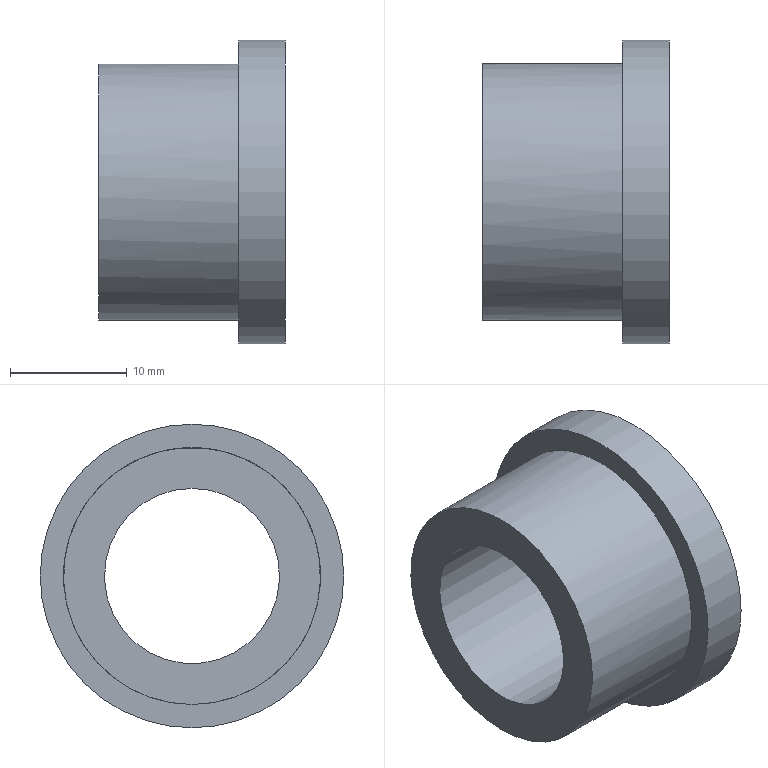Component | NX | LOCATING_BUSH | 1 solid | 6 faces | box 16 x 26 x 26 mm | volume 3858 mm3 | plane 3 | cylinder 3 | commonest cylinder face diameters 22 x1 26 x1 15 x1
STEP:
#1=CARTESIAN_POINT('',(0.,0.,0.));
#2=DIRECTION('',(0.,0.,1.));
#3=DIRECTION('',(1.,0.,0.));
#4=AXIS2_PLACEMENT_3D('',#1,#2,#3);
#5=CARTESIAN_POINT('',(-30.772,-17.527,-251.219));
#6=VERTEX_POINT('',#5);
#7=CARTESIAN_POINT('',(-30.772,-17.527,-258.719));
#8=DIRECTION('',(-1.,0.,0.));
#9=DIRECTION('',(0.,0.,1.));
#10=AXIS2_PLACEMENT_3D('',#7,#8,#9);
#11=CIRCLE('',#10,7.5);
#12=CARTESIAN_POINT('',(-30.772,-17.527,-258.719));
#13=DIRECTION('',(-1.,0.,0.));
#14=DIRECTION('',(0.,0.,1.));
#15=AXIS2_PLACEMENT_3D('',#12,#13,#14);
#16=PLANE('',#15);
#17=CARTESIAN_POINT('',(0.,0.));
#18=DIRECTION('',(1.,0.));
#19=AXIS2_PLACEMENT_2D('',#17,#18);
#20=CIRCLE('',#19,7.5);
#21=(GEOMETRIC_REPRESENTATION_CONTEXT(2)PARAMETRIC_REPRESENTATION_CONTEXT()REPRESENTATION_CONTEXT('',''));
#22=DEFINITIONAL_REPRESENTATION('',(#20),#21);
#23=PCURVE('',#16,#22);
#24=CARTESIAN_POINT('',(-14.772,-17.527,-258.719));
#25=DIRECTION('',(-1.,0.,0.));
#26=DIRECTION('',(0.,0.,1.));
#27=AXIS2_PLACEMENT_3D('',#24,#25,#26);
#28=CYLINDRICAL_SURFACE('',#27,7.5);
#29=CARTESIAN_POINT('',(0.,16.));
#30=DIRECTION('',(1.,0.));
#31=VECTOR('',#30,1.);
#32=LINE('',#29,#31);
#33=(GEOMETRIC_REPRESENTATION_CONTEXT(2)PARAMETRIC_REPRESENTATION_CONTEXT()REPRESENTATION_CONTEXT('',''));
#34=DEFINITIONAL_REPRESENTATION('',(#32),#33);
#35=PCURVE('',#28,#34);
#36=SURFACE_CURVE('',#11,(#23,#35),.PCURVE_S1.);
#37=EDGE_CURVE('',#6,#6,#36,.T.);
#38=ORIENTED_EDGE('',*,*,#37,.F.);
#39=EDGE_LOOP('',(#38));
#40=FACE_BOUND('',#39,.T.);
#41=CARTESIAN_POINT('',(-30.772,-17.527,-269.719));
#42=VERTEX_POINT('',#41);
#43=CARTESIAN_POINT('',(-30.772,-17.527,-258.719));
#44=DIRECTION('',(1.,0.,0.));
#45=DIRECTION('',(0.,0.,-1.));
#46=AXIS2_PLACEMENT_3D('',#43,#44,#45);
#47=CIRCLE('',#46,11.);
#48=CARTESIAN_POINT('',(-11.,0.));
#49=CARTESIAN_POINT('',(-11.,19.053));
#50=CARTESIAN_POINT('',(5.5,9.526));
#51=CARTESIAN_POINT('',(22.,0.));
#52=CARTESIAN_POINT('',(5.5,-9.526));
#53=CARTESIAN_POINT('',(-11.,-19.053));
#54=CARTESIAN_POINT('',(-11.,0.));
#55=(BOUNDED_CURVE()B_SPLINE_CURVE(2,(#48,#49,#50,#51,#52,#53,#54),.UNSPECIFIED.,.T.,.F.)B_SPLINE_CURVE_WITH_KNOTS((1,2,2,2,2,1),(-2.094,0.,2.094,4.189,6.283,8.378),.UNSPECIFIED.)CURVE()GEOMETRIC_REPRESENTATION_ITEM()RATIONAL_B_SPLINE_CURVE((1.,0.5,1.,0.5,1.,0.5,1.))REPRESENTATION_ITEM(''));
#56=(GEOMETRIC_REPRESENTATION_CONTEXT(2)PARAMETRIC_REPRESENTATION_CONTEXT()REPRESENTATION_CONTEXT('',''));
#57=DEFINITIONAL_REPRESENTATION('',(#55),#56);
#58=PCURVE('',#16,#57);
#59=CARTESIAN_POINT('',(-30.772,-17.527,-258.719));
#60=DIRECTION('',(1.,0.,0.));
#61=DIRECTION('',(0.,0.,-1.));
#62=AXIS2_PLACEMENT_3D('',#59,#60,#61);
#63=CYLINDRICAL_SURFACE('',#62,11.);
#64=CARTESIAN_POINT('',(0.,0.));
#65=DIRECTION('',(1.,0.));
#66=VECTOR('',#65,1.);
#67=LINE('',#64,#66);
#68=(GEOMETRIC_REPRESENTATION_CONTEXT(2)PARAMETRIC_REPRESENTATION_CONTEXT()REPRESENTATION_CONTEXT('',''));
#69=DEFINITIONAL_REPRESENTATION('',(#67),#68);
#70=PCURVE('',#63,#69);
#71=SURFACE_CURVE('',#47,(#58,#70),.PCURVE_S1.);
#72=EDGE_CURVE('',#42,#42,#71,.T.);
#73=ORIENTED_EDGE('',*,*,#72,.F.);
#74=EDGE_LOOP('',(#73));
#75=FACE_BOUND('',#74,.T.);
#76=ADVANCED_FACE('',(#40,#75),#16,.T.);
#77=CARTESIAN_POINT('',(-18.772,-17.527,-269.719));
#78=VERTEX_POINT('',#77);
#79=CARTESIAN_POINT('',(-18.772,-17.527,-247.719));
#80=VERTEX_POINT('',#79);
#81=CARTESIAN_POINT('',(-18.772,-17.527,-258.719));
#82=DIRECTION('',(1.,0.,0.));
#83=DIRECTION('',(0.,0.,1.));
#84=AXIS2_PLACEMENT_3D('',#81,#82,#83);
#85=CIRCLE('',#84,11.);
#86=CARTESIAN_POINT('',(-3.142,12.));
#87=DIRECTION('',(1.,0.));
#88=VECTOR('',#87,1.);
#89=LINE('',#86,#88);
#90=(GEOMETRIC_REPRESENTATION_CONTEXT(2)PARAMETRIC_REPRESENTATION_CONTEXT()REPRESENTATION_CONTEXT('',''));
#91=DEFINITIONAL_REPRESENTATION('',(#89),#90);
#92=PCURVE('',#63,#91);
#93=CARTESIAN_POINT('',(-18.772,-17.527,-258.719));
#94=DIRECTION('',(-1.,0.,0.));
#95=DIRECTION('',(0.,0.,1.));
#96=AXIS2_PLACEMENT_3D('',#93,#94,#95);
#97=PLANE('',#96);
#98=CARTESIAN_POINT('',(11.,0.));
#99=CARTESIAN_POINT('',(11.,-19.053));
#100=CARTESIAN_POINT('',(-5.5,-9.526));
#101=CARTESIAN_POINT('',(-22.,-0.));
#102=CARTESIAN_POINT('',(-5.5,9.526));
#103=CARTESIAN_POINT('',(11.,19.053));
#104=CARTESIAN_POINT('',(11.,0.));
#105=(BOUNDED_CURVE()B_SPLINE_CURVE(2,(#98,#99,#100,#101,#102,#103,#104),.UNSPECIFIED.,.T.,.F.)B_SPLINE_CURVE_WITH_KNOTS((1,2,2,2,2,1),(-2.094,0.,2.094,4.189,6.283,8.378),.UNSPECIFIED.)CURVE()GEOMETRIC_REPRESENTATION_ITEM()RATIONAL_B_SPLINE_CURVE((1.,0.5,1.,0.5,1.,0.5,1.))REPRESENTATION_ITEM(''));
#106=(GEOMETRIC_REPRESENTATION_CONTEXT(2)PARAMETRIC_REPRESENTATION_CONTEXT()REPRESENTATION_CONTEXT('',''));
#107=DEFINITIONAL_REPRESENTATION('',(#105),#106);
#108=PCURVE('',#97,#107);
#109=SURFACE_CURVE('',#85,(#92,#108),.PCURVE_S1.);
#110=EDGE_CURVE('',#78,#80,#109,.T.);
#111=ORIENTED_EDGE('',*,*,#110,.F.);
#112=CARTESIAN_POINT('',(-30.772,-17.527,-269.719));
#113=CARTESIAN_POINT('',(-18.772,-17.527,-269.719));
#114=B_SPLINE_CURVE_WITH_KNOTS('',1,(#112,#113),.UNSPECIFIED.,.F.,.F.,(2,2),(0.,12.),.PIECEWISE_BEZIER_KNOTS.);
#115=CARTESIAN_POINT('',(0.,0.));
#116=DIRECTION('',(0.,1.));
#117=VECTOR('',#116,1.);
#118=LINE('',#115,#117);
#119=(GEOMETRIC_REPRESENTATION_CONTEXT(2)PARAMETRIC_REPRESENTATION_CONTEXT()REPRESENTATION_CONTEXT('',''));
#120=DEFINITIONAL_REPRESENTATION('',(#118),#119);
#121=PCURVE('',#63,#120);
#122=CARTESIAN_POINT('',(6.283,0.));
#123=DIRECTION('',(0.,1.));
#124=VECTOR('',#123,1.);
#125=LINE('',#122,#124);
#126=(GEOMETRIC_REPRESENTATION_CONTEXT(2)PARAMETRIC_REPRESENTATION_CONTEXT()REPRESENTATION_CONTEXT('',''));
#127=DEFINITIONAL_REPRESENTATION('',(#125),#126);
#128=PCURVE('',#63,#127);
#129=SEAM_CURVE('',#114,(#121,#128),.PCURVE_S1.);
#130=EDGE_CURVE('',#42,#78,#129,.T.);
#131=ORIENTED_EDGE('',*,*,#130,.F.);
#132=ORIENTED_EDGE('',*,*,#72,.T.);
#133=ORIENTED_EDGE('',*,*,#130,.T.);
#134=CARTESIAN_POINT('',(-18.772,-17.527,-258.719));
#135=DIRECTION('',(1.,0.,0.));
#136=DIRECTION('',(0.,0.,1.));
#137=AXIS2_PLACEMENT_3D('',#134,#135,#136);
#138=CIRCLE('',#137,11.);
#139=CARTESIAN_POINT('',(3.142,12.));
#140=DIRECTION('',(1.,0.));
#141=VECTOR('',#140,1.);
#142=LINE('',#139,#141);
#143=(GEOMETRIC_REPRESENTATION_CONTEXT(2)PARAMETRIC_REPRESENTATION_CONTEXT()REPRESENTATION_CONTEXT('',''));
#144=DEFINITIONAL_REPRESENTATION('',(#142),#143);
#145=PCURVE('',#63,#144);
#146=CARTESIAN_POINT('',(11.,0.));
#147=CARTESIAN_POINT('',(11.,-19.053));
#148=CARTESIAN_POINT('',(-5.5,-9.526));
#149=CARTESIAN_POINT('',(-22.,-0.));
#150=CARTESIAN_POINT('',(-5.5,9.526));
#151=CARTESIAN_POINT('',(11.,19.053));
#152=CARTESIAN_POINT('',(11.,0.));
#153=(BOUNDED_CURVE()B_SPLINE_CURVE(2,(#146,#147,#148,#149,#150,#151,#152),.UNSPECIFIED.,.T.,.F.)B_SPLINE_CURVE_WITH_KNOTS((1,2,2,2,2,1),(-2.094,0.,2.094,4.189,6.283,8.378),.UNSPECIFIED.)CURVE()GEOMETRIC_REPRESENTATION_ITEM()RATIONAL_B_SPLINE_CURVE((1.,0.5,1.,0.5,1.,0.5,1.))REPRESENTATION_ITEM(''));
#154=(GEOMETRIC_REPRESENTATION_CONTEXT(2)PARAMETRIC_REPRESENTATION_CONTEXT()REPRESENTATION_CONTEXT('',''));
#155=DEFINITIONAL_REPRESENTATION('',(#153),#154);
#156=PCURVE('',#97,#155);
#157=SURFACE_CURVE('',#138,(#145,#156),.PCURVE_S1.);
#158=EDGE_CURVE('',#80,#78,#157,.T.);
#159=ORIENTED_EDGE('',*,*,#158,.F.);
#160=EDGE_LOOP('',(#111,#131,#132,#133,#159));
#161=FACE_BOUND('',#160,.T.);
#162=ADVANCED_FACE('',(#161),#63,.T.);
#163=CARTESIAN_POINT('',(-14.772,-17.527,-251.219));
#164=VERTEX_POINT('',#163);
#165=CARTESIAN_POINT('',(-14.772,-17.527,-258.719));
#166=DIRECTION('',(-1.,0.,0.));
#167=DIRECTION('',(0.,0.,1.));
#168=AXIS2_PLACEMENT_3D('',#165,#166,#167);
#169=CIRCLE('',#168,7.5);
#170=CARTESIAN_POINT('',(-14.772,-17.527,-258.719));
#171=DIRECTION('',(1.,0.,0.));
#172=DIRECTION('',(0.,0.,-1.));
#173=AXIS2_PLACEMENT_3D('',#170,#171,#172);
#174=PLANE('',#173);
#175=CARTESIAN_POINT('',(-7.5,0.));
#176=CARTESIAN_POINT('',(-7.5,12.99));
#177=CARTESIAN_POINT('',(3.75,6.495));
#178=CARTESIAN_POINT('',(15.,0.));
#179=CARTESIAN_POINT('',(3.75,-6.495));
#180=CARTESIAN_POINT('',(-7.5,-12.99));
#181=CARTESIAN_POINT('',(-7.5,0.));
#182=(BOUNDED_CURVE()B_SPLINE_CURVE(2,(#175,#176,#177,#178,#179,#180,#181),.UNSPECIFIED.,.T.,.F.)B_SPLINE_CURVE_WITH_KNOTS((1,2,2,2,2,1),(-2.094,0.,2.094,4.189,6.283,8.378),.UNSPECIFIED.)CURVE()GEOMETRIC_REPRESENTATION_ITEM()RATIONAL_B_SPLINE_CURVE((1.,0.5,1.,0.5,1.,0.5,1.))REPRESENTATION_ITEM(''));
#183=(GEOMETRIC_REPRESENTATION_CONTEXT(2)PARAMETRIC_REPRESENTATION_CONTEXT()REPRESENTATION_CONTEXT('',''));
#184=DEFINITIONAL_REPRESENTATION('',(#182),#183);
#185=PCURVE('',#174,#184);
#186=CARTESIAN_POINT('',(0.,0.));
#187=DIRECTION('',(1.,0.));
#188=VECTOR('',#187,1.);
#189=LINE('',#186,#188);
#190=(GEOMETRIC_REPRESENTATION_CONTEXT(2)PARAMETRIC_REPRESENTATION_CONTEXT()REPRESENTATION_CONTEXT('',''));
#191=DEFINITIONAL_REPRESENTATION('',(#189),#190);
#192=PCURVE('',#28,#191);
#193=SURFACE_CURVE('',#169,(#185,#192),.PCURVE_S1.);
#194=EDGE_CURVE('',#164,#164,#193,.T.);
#195=ORIENTED_EDGE('',*,*,#194,.T.);
#196=EDGE_LOOP('',(#195));
#197=FACE_BOUND('',#196,.T.);
#198=CARTESIAN_POINT('',(-14.772,-17.527,-271.719));
#199=VERTEX_POINT('',#198);
#200=CARTESIAN_POINT('',(-14.772,-17.527,-258.719));
#201=DIRECTION('',(-1.,0.,0.));
#202=DIRECTION('',(0.,0.,-1.));
#203=AXIS2_PLACEMENT_3D('',#200,#201,#202);
#204=CIRCLE('',#203,13.);
#205=CARTESIAN_POINT('',(13.,0.));
#206=CARTESIAN_POINT('',(13.,-22.517));
#207=CARTESIAN_POINT('',(-6.5,-11.258));
#208=CARTESIAN_POINT('',(-26.,-0.));
#209=CARTESIAN_POINT('',(-6.5,11.258));
#210=CARTESIAN_POINT('',(13.,22.517));
#211=CARTESIAN_POINT('',(13.,0.));
#212=(BOUNDED_CURVE()B_SPLINE_CURVE(2,(#205,#206,#207,#208,#209,#210,#211),.UNSPECIFIED.,.T.,.F.)B_SPLINE_CURVE_WITH_KNOTS((1,2,2,2,2,1),(-2.094,0.,2.094,4.189,6.283,8.378),.UNSPECIFIED.)CURVE()GEOMETRIC_REPRESENTATION_ITEM()RATIONAL_B_SPLINE_CURVE((1.,0.5,1.,0.5,1.,0.5,1.))REPRESENTATION_ITEM(''));
#213=(GEOMETRIC_REPRESENTATION_CONTEXT(2)PARAMETRIC_REPRESENTATION_CONTEXT()REPRESENTATION_CONTEXT('',''));
#214=DEFINITIONAL_REPRESENTATION('',(#212),#213);
#215=PCURVE('',#174,#214);
#216=CARTESIAN_POINT('',(-18.772,-17.527,-258.719));
#217=DIRECTION('',(1.,0.,0.));
#218=DIRECTION('',(0.,0.,-1.));
#219=AXIS2_PLACEMENT_3D('',#216,#217,#218);
#220=CYLINDRICAL_SURFACE('',#219,13.);
#221=CARTESIAN_POINT('',(6.283,4.));
#222=DIRECTION('',(-1.,0.));
#223=VECTOR('',#222,1.);
#224=LINE('',#221,#223);
#225=(GEOMETRIC_REPRESENTATION_CONTEXT(2)PARAMETRIC_REPRESENTATION_CONTEXT()REPRESENTATION_CONTEXT('',''));
#226=DEFINITIONAL_REPRESENTATION('',(#224),#225);
#227=PCURVE('',#220,#226);
#228=SURFACE_CURVE('',#204,(#215,#227),.PCURVE_S1.);
#229=EDGE_CURVE('',#199,#199,#228,.T.);
#230=ORIENTED_EDGE('',*,*,#229,.F.);
#231=EDGE_LOOP('',(#230));
#232=FACE_BOUND('',#231,.T.);
#233=ADVANCED_FACE('',(#197,#232),#174,.T.);
#234=ORIENTED_EDGE('',*,*,#158,.T.);
#235=ORIENTED_EDGE('',*,*,#110,.T.);
#236=EDGE_LOOP('',(#234,#235));
#237=FACE_BOUND('',#236,.T.);
#238=CARTESIAN_POINT('',(-18.772,-17.527,-271.719));
#239=VERTEX_POINT('',#238);
#240=CARTESIAN_POINT('',(-18.772,-17.527,-258.719));
#241=DIRECTION('',(1.,0.,0.));
#242=DIRECTION('',(0.,0.,-1.));
#243=AXIS2_PLACEMENT_3D('',#240,#241,#242);
#244=CIRCLE('',#243,13.);
#245=CARTESIAN_POINT('',(-13.,0.));
#246=CARTESIAN_POINT('',(-13.,22.517));
#247=CARTESIAN_POINT('',(6.5,11.258));
#248=CARTESIAN_POINT('',(26.,0.));
#249=CARTESIAN_POINT('',(6.5,-11.258));
#250=CARTESIAN_POINT('',(-13.,-22.517));
#251=CARTESIAN_POINT('',(-13.,0.));
#252=(BOUNDED_CURVE()B_SPLINE_CURVE(2,(#245,#246,#247,#248,#249,#250,#251),.UNSPECIFIED.,.T.,.F.)B_SPLINE_CURVE_WITH_KNOTS((1,2,2,2,2,1),(-2.094,0.,2.094,4.189,6.283,8.378),.UNSPECIFIED.)CURVE()GEOMETRIC_REPRESENTATION_ITEM()RATIONAL_B_SPLINE_CURVE((1.,0.5,1.,0.5,1.,0.5,1.))REPRESENTATION_ITEM(''));
#253=(GEOMETRIC_REPRESENTATION_CONTEXT(2)PARAMETRIC_REPRESENTATION_CONTEXT()REPRESENTATION_CONTEXT('',''));
#254=DEFINITIONAL_REPRESENTATION('',(#252),#253);
#255=PCURVE('',#97,#254);
#256=CARTESIAN_POINT('',(0.,0.));
#257=DIRECTION('',(1.,0.));
#258=VECTOR('',#257,1.);
#259=LINE('',#256,#258);
#260=(GEOMETRIC_REPRESENTATION_CONTEXT(2)PARAMETRIC_REPRESENTATION_CONTEXT()REPRESENTATION_CONTEXT('',''));
#261=DEFINITIONAL_REPRESENTATION('',(#259),#260);
#262=PCURVE('',#220,#261);
#263=SURFACE_CURVE('',#244,(#255,#262),.PCURVE_S1.);
#264=EDGE_CURVE('',#239,#239,#263,.T.);
#265=ORIENTED_EDGE('',*,*,#264,.F.);
#266=EDGE_LOOP('',(#265));
#267=FACE_BOUND('',#266,.T.);
#268=ADVANCED_FACE('',(#237,#267),#97,.T.);
#269=ORIENTED_EDGE('',*,*,#229,.T.);
#270=CARTESIAN_POINT('',(-18.772,-17.527,-271.719));
#271=CARTESIAN_POINT('',(-14.772,-17.527,-271.719));
#272=B_SPLINE_CURVE_WITH_KNOTS('',1,(#270,#271),.UNSPECIFIED.,.F.,.F.,(2,2),(0.,4.),.PIECEWISE_BEZIER_KNOTS.);
#273=CARTESIAN_POINT('',(0.,0.));
#274=DIRECTION('',(0.,1.));
#275=VECTOR('',#274,1.);
#276=LINE('',#273,#275);
#277=(GEOMETRIC_REPRESENTATION_CONTEXT(2)PARAMETRIC_REPRESENTATION_CONTEXT()REPRESENTATION_CONTEXT('',''));
#278=DEFINITIONAL_REPRESENTATION('',(#276),#277);
#279=PCURVE('',#220,#278);
#280=CARTESIAN_POINT('',(6.283,0.));
#281=DIRECTION('',(0.,1.));
#282=VECTOR('',#281,1.);
#283=LINE('',#280,#282);
#284=(GEOMETRIC_REPRESENTATION_CONTEXT(2)PARAMETRIC_REPRESENTATION_CONTEXT()REPRESENTATION_CONTEXT('',''));
#285=DEFINITIONAL_REPRESENTATION('',(#283),#284);
#286=PCURVE('',#220,#285);
#287=SEAM_CURVE('',#272,(#279,#286),.PCURVE_S1.);
#288=EDGE_CURVE('',#239,#199,#287,.T.);
#289=ORIENTED_EDGE('',*,*,#288,.F.);
#290=ORIENTED_EDGE('',*,*,#264,.T.);
#291=ORIENTED_EDGE('',*,*,#288,.T.);
#292=EDGE_LOOP('',(#269,#289,#290,#291));
#293=FACE_BOUND('',#292,.T.);
#294=ADVANCED_FACE('',(#293),#220,.T.);
#295=ORIENTED_EDGE('',*,*,#37,.F.);
#296=CARTESIAN_POINT('',(-14.772,-17.527,-251.219));
#297=CARTESIAN_POINT('',(-30.772,-17.527,-251.219));
#298=B_SPLINE_CURVE_WITH_KNOTS('',1,(#296,#297),.UNSPECIFIED.,.F.,.F.,(2,2),(0.,16.),.PIECEWISE_BEZIER_KNOTS.);
#299=CARTESIAN_POINT('',(0.,0.));
#300=DIRECTION('',(0.,1.));
#301=VECTOR('',#300,1.);
#302=LINE('',#299,#301);
#303=(GEOMETRIC_REPRESENTATION_CONTEXT(2)PARAMETRIC_REPRESENTATION_CONTEXT()REPRESENTATION_CONTEXT('',''));
#304=DEFINITIONAL_REPRESENTATION('',(#302),#303);
#305=PCURVE('',#28,#304);
#306=CARTESIAN_POINT('',(6.283,0.));
#307=DIRECTION('',(0.,1.));
#308=VECTOR('',#307,1.);
#309=LINE('',#306,#308);
#310=(GEOMETRIC_REPRESENTATION_CONTEXT(2)PARAMETRIC_REPRESENTATION_CONTEXT()REPRESENTATION_CONTEXT('',''));
#311=DEFINITIONAL_REPRESENTATION('',(#309),#310);
#312=PCURVE('',#28,#311);
#313=SEAM_CURVE('',#298,(#305,#312),.PCURVE_S1.);
#314=EDGE_CURVE('',#164,#6,#313,.T.);
#315=ORIENTED_EDGE('',*,*,#314,.F.);
#316=ORIENTED_EDGE('',*,*,#194,.T.);
#317=ORIENTED_EDGE('',*,*,#314,.T.);
#318=EDGE_LOOP('',(#295,#315,#316,#317));
#319=FACE_BOUND('',#318,.F.);
#320=ADVANCED_FACE('',(#319),#28,.F.);
#321=CLOSED_SHELL('',(#76,#162,#233,#268,#294,#320));
#322=MANIFOLD_SOLID_BREP('',#321);
#323=(LENGTH_UNIT()NAMED_UNIT(*)SI_UNIT(.MILLI.,.METRE.));
#324=UNCERTAINTY_MEASURE_WITH_UNIT(LENGTH_MEASURE(0.000005),#323,'','');
#325=(NAMED_UNIT(*)PLANE_ANGLE_UNIT()SI_UNIT($,.RADIAN.));
#326=(NAMED_UNIT(*)SI_UNIT($,.STERADIAN.)SOLID_ANGLE_UNIT());
#327=(GEOMETRIC_REPRESENTATION_CONTEXT(3)GLOBAL_UNCERTAINTY_ASSIGNED_CONTEXT((#324))GLOBAL_UNIT_ASSIGNED_CONTEXT((#323,#325,#326))REPRESENTATION_CONTEXT('',''));
#328=ADVANCED_BREP_SHAPE_REPRESENTATION('',(#4,#322),#327);